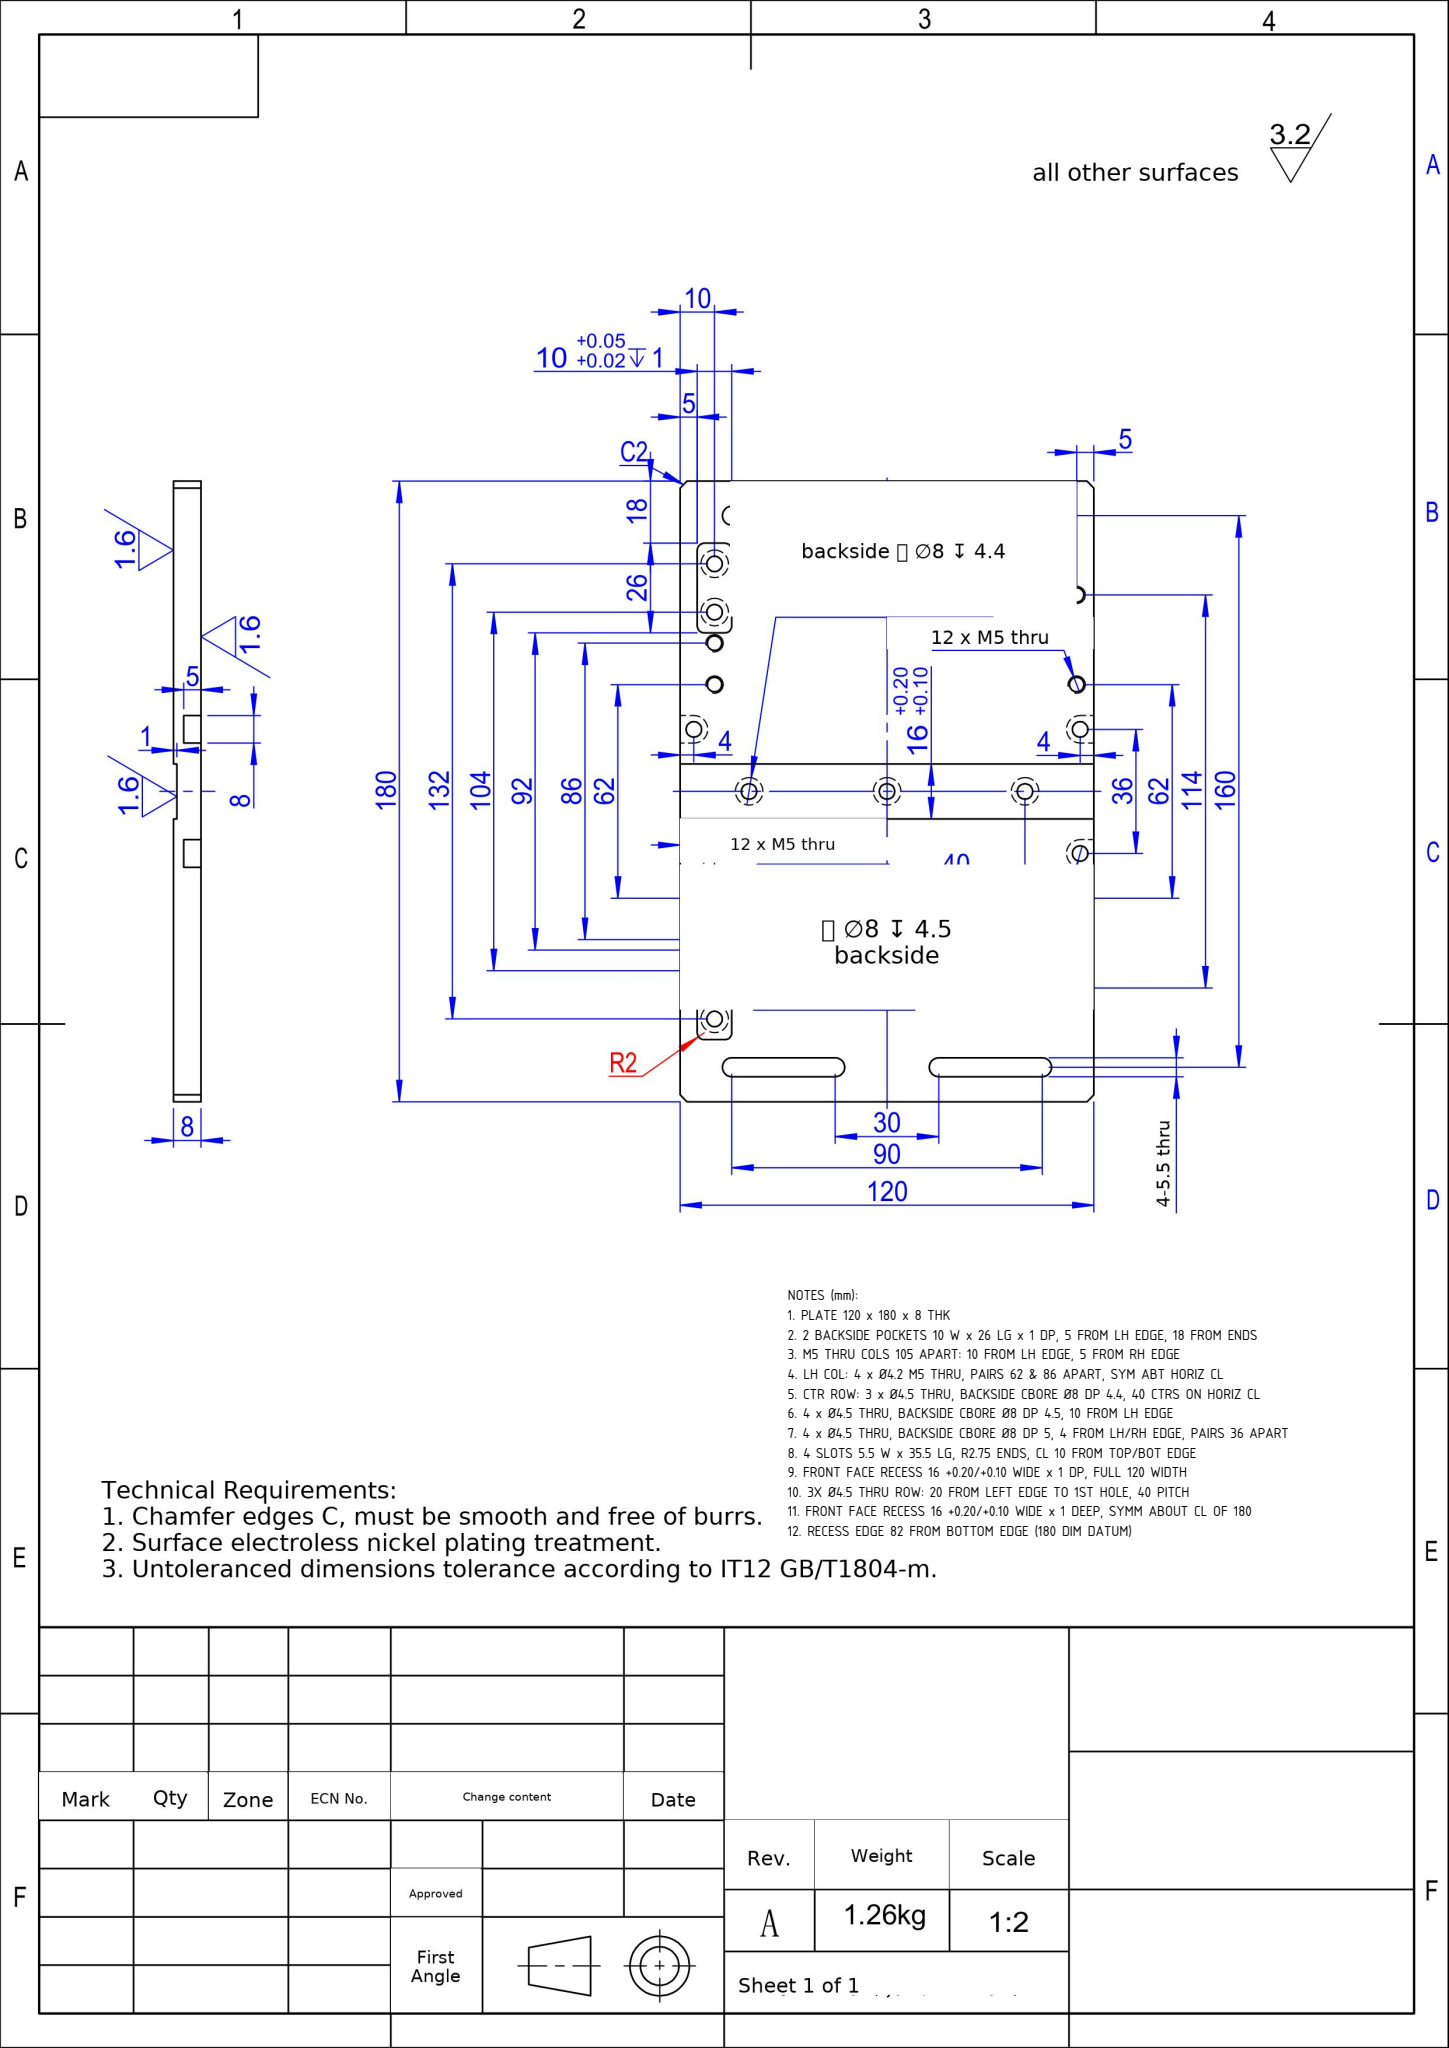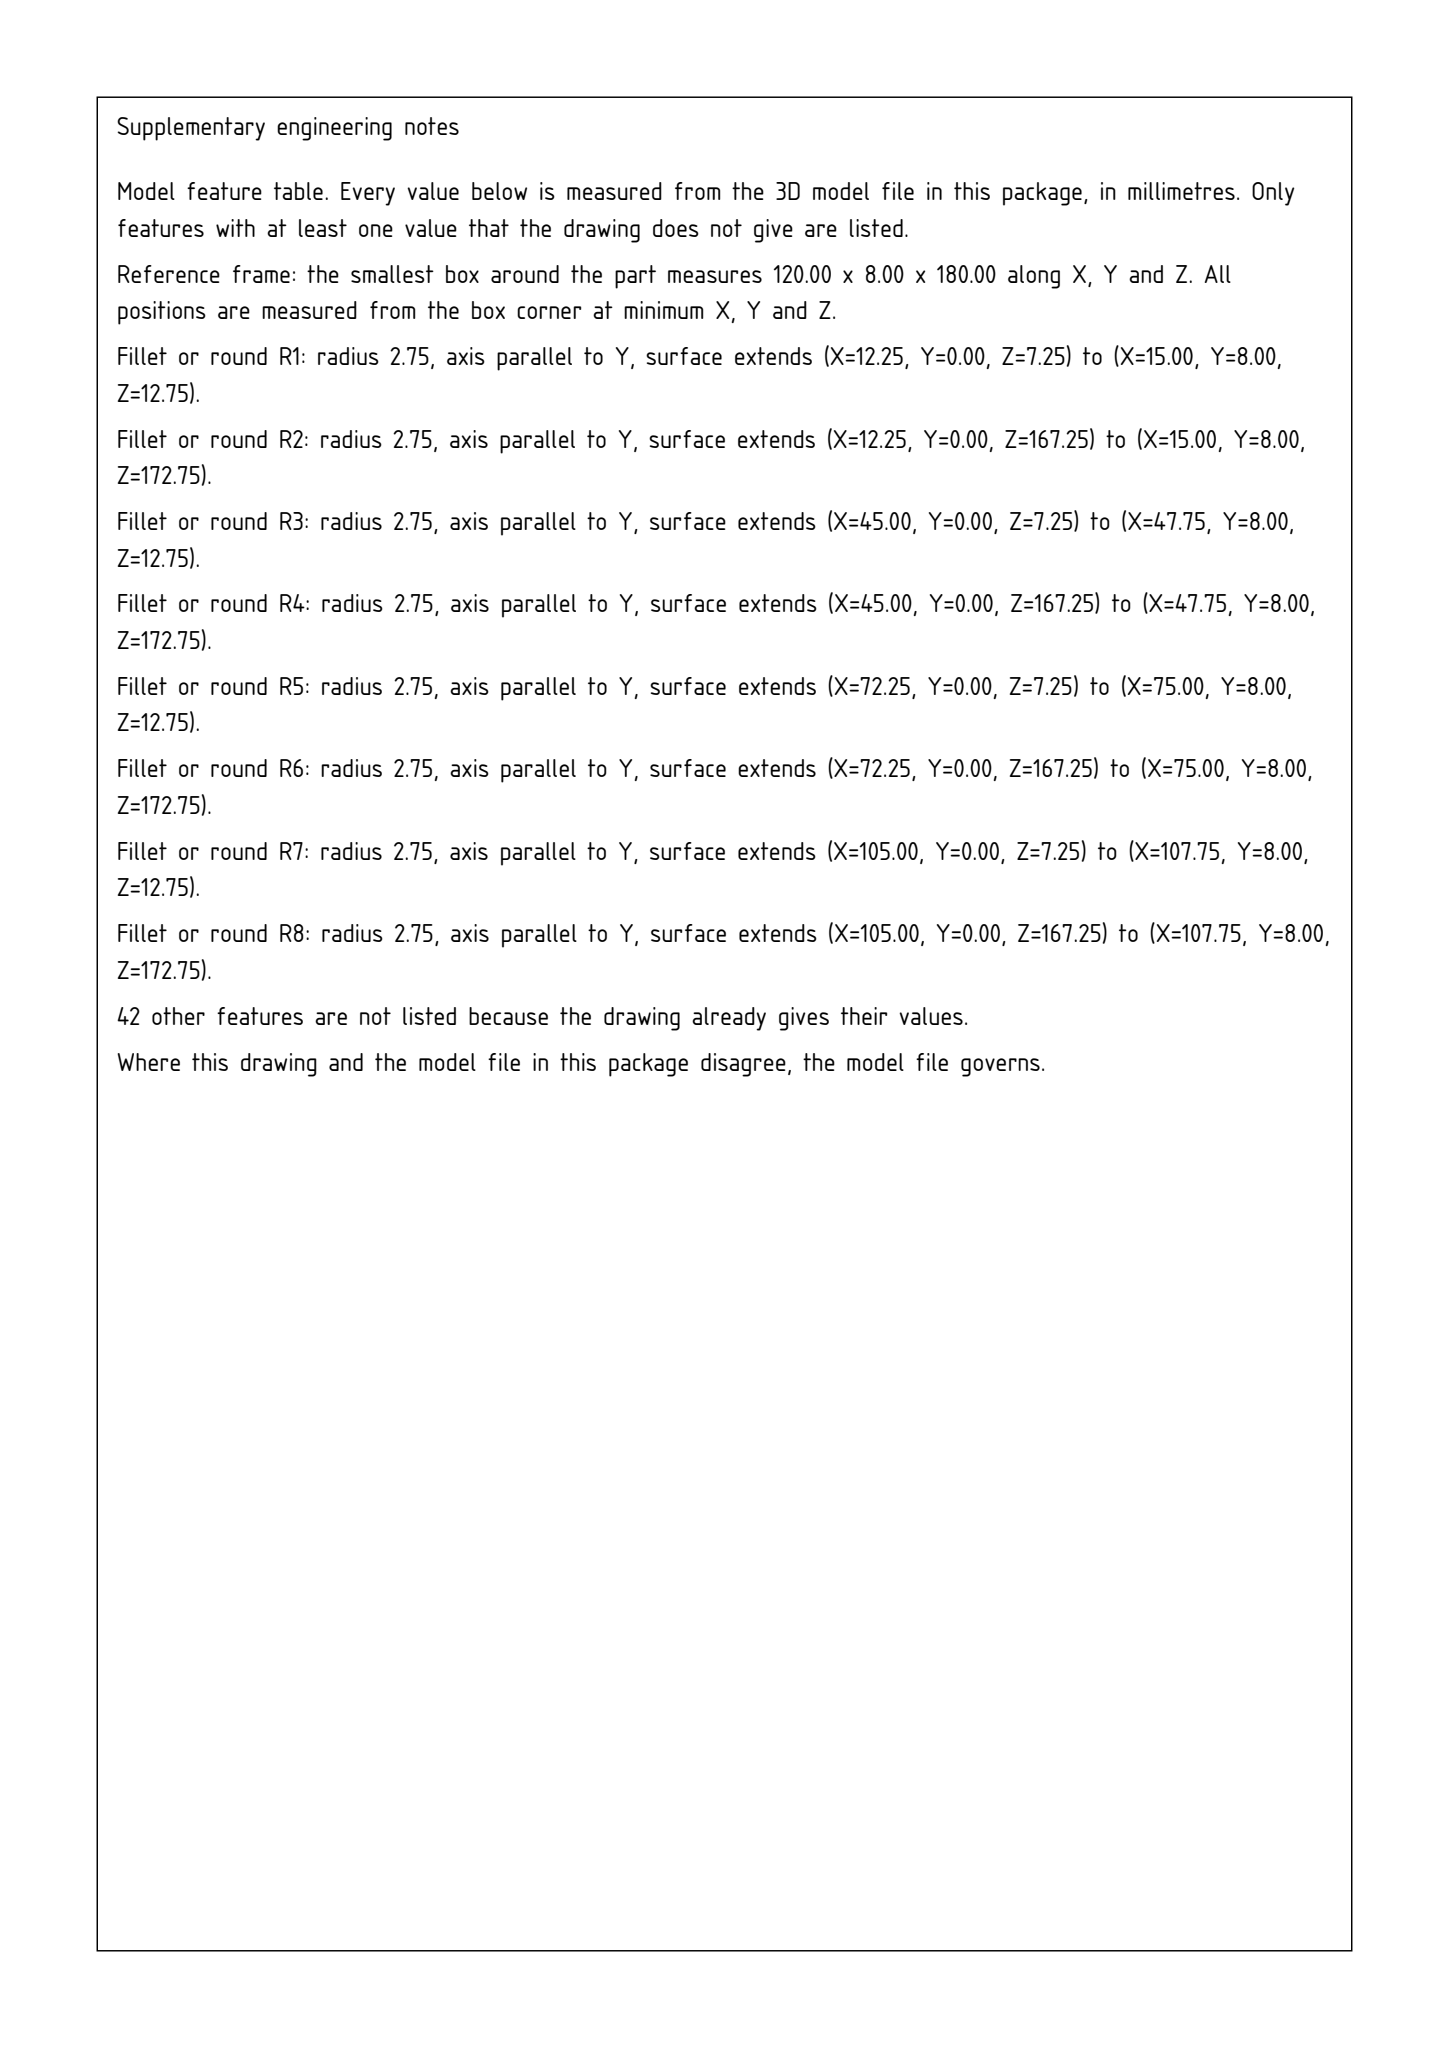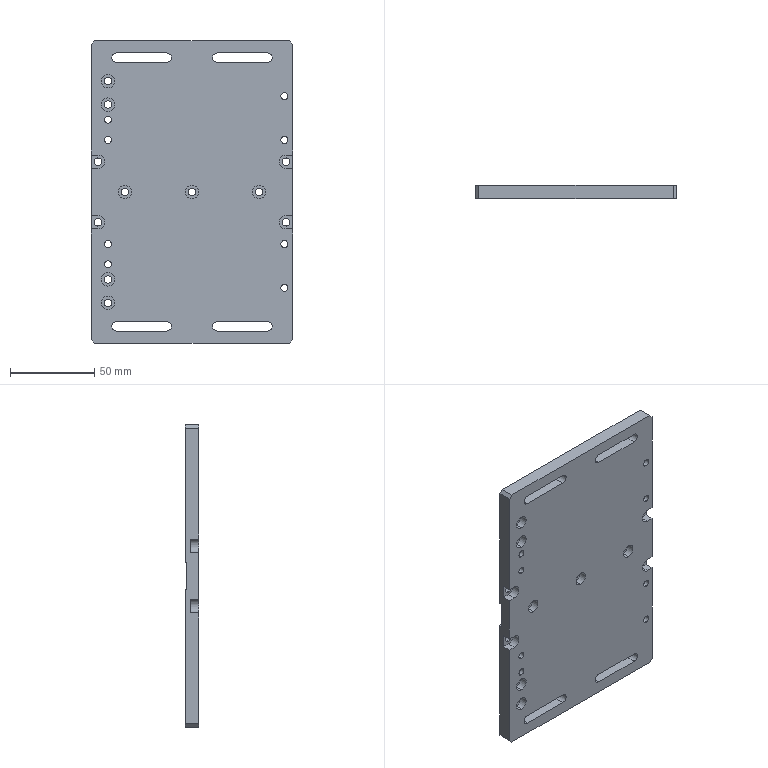Part | SolidWorks | mm | 1 solid | 123 faces | box 120 x 8 x 180 mm | volume 160191 mm3 | cylinder 72 | plane 51 | commonest cylinder face diameters 4.5 x22 8 x18 4.2 x16 4 x8 5.5 x8
Drawing notes:
PLATE 120 x 180 x 8 THK | from the solid: bbox_xyz 120 x 8 x 180
2 BACKSIDE POCKETS 10 W x 26 LG x 1 DP, 5 FROM LH EDGE, 18 FROM ENDS | from the solid: x planes 5 & 15 (10 wide); y 7.0 vs 8.0 face = 1 DP; z 18-44 & 136-162 (26 lg, 18 from ends)
M5 THRU COLS 105 APART: 10 FROM LH EDGE, 5 FROM RH EDGE | from the solid: Ø4.2 thru cols at x=10 and x=115; 115-10=105; 120-115=5
LH COL: 4 x Ø4.2 M5 THRU, PAIRS 62 & 86 APART, SYM ABT HORIZ CL | from the solid: Ø4.2 thru (len 8) at x=10, z=47/59/121/133; 59-121=62, 47-133=86, sym about z=90
CTR ROW: 3 x Ø4.5 THRU, BACKSIDE CBORE Ø8 DP 4.4, 40 CTRS ON HORIZ CL | from the solid: Ø4.5 at x=20,60,100 (40 spacing), z=90=180/2; Ø8 cbore len 4.4 same axes
4 x Ø4.5 THRU, BACKSIDE CBORE Ø8 DP 4.5, 10 FROM LH EDGE | from the solid: Ø4.5 y-holes at x=10, z=24,38,142,156 with Ø8 cbore len 4.5
4 x Ø4.5 THRU, BACKSIDE CBORE Ø8 DP 5, 4 FROM LH/RH EDGE, PAIRS 36 APART | from the solid: Ø4.5 at x=4 & 116, z=72 & 108 (36 apart, sym abt z=90); Ø8 cbore len 5
4 SLOTS 5.5 W x 35.5 LG, R2.75 ENDS, CL 10 FROM TOP/BOT EDGE | from the solid: Ø5.5 thru ends x=15/45 & 75/105 at z=10 and z=170; z planes 7.25/12.75 & 167.25/172.75
FRONT FACE RECESS 16 +0.20/+0.10 WIDE x 1 DP, FULL 120 WIDTH | from the solid: Z planes 82 & 98 (16 apart), Y plane 7.0 vs front face Y=8.0 -> 1 deep; spans X 0-120 (bbox width)
3X Ø4.5 THRU ROW: 20 FROM LEFT EDGE TO 1ST HOLE, 40 PITCH | from the solid: Ø4.5 holes at X=20, 60, 100 (Z=90); left edge X=0; middle hole on part CL X=60
FRONT FACE RECESS 16 +0.20/+0.10 WIDE x 1 DEEP, SYMM ABOUT CL OF 180 | from the solid: z-planes 82 & 98 bound 16 wide slot, centred at z=90 = 180/2; depth 1 (y 7.0 to 8.0), full 120 width
RECESS EDGE 82 FROM BOTTOM EDGE (180 DIM DATUM) | from the solid: z=82 and z=98 planes on 180 length from z=0 edge
build123d program:
from build123d import *

# Parameters (mm, degrees)
SKETCH1_W                                       = 120
SKETCH1_H                                       = 180
BOSS_EXTRUDE1_DEPTH                             = 8
SKETCH2_W                                       = 120
SKETCH2_H                                       = 16
CUT_EXTRUDE1_DEPTH                              = 1
M4_HEX_SOCKET_HEAD_CAP_SCREW_CBORE2_D           = 4.5
M4_HEX_SOCKET_HEAD_CAP_SCREW_CBORE2_CBORE_D     = 8
M4_HEX_SOCKET_HEAD_CAP_SCREW_CBORE2_CBORE_DEPTH = 4.4
M4_HEX_SOCKET_HEAD_CAP_SCREW_CBORE1_D           = 4.5
M4_HEX_SOCKET_HEAD_CAP_SCREW_CBORE1_CBORE_D     = 8
M4_HEX_SOCKET_HEAD_CAP_SCREW_CBORE1_CBORE_DEPTH = 4.5
SKETCH21_W                                      = 10
SKETCH21_H                                      = 26
CUT_EXTRUDE5_DEPTH                              = 1
FILLET2_R                                       = 2
CUT_EXTRUDE2_DEPTH                              = 109.462
FILLET2_OF_MIRROR1_R                            = 2
CHAMFER1_SIZE                                   = 2
MIRROR9_COPY_1_DEPTH                            = 109.462
LPATTERN3_COUNT                                 = 3
LPATTERN3_PITCH                                 = 40
M5_TAPPED_HOLE1_D                               = 4.2
M5_TAPPED_HOLE2_D                               = 4.2
M4_CLEARANCE_HOLE1_D                            = 4.5
CUT_EXTRUDE4_DEPTH                              = 5


with BuildPart() as part:
    # Sketch1 → Boss-Extrude1 (new body)
    with BuildSketch(Plane(origin=(0, 0, 0), x_dir=(1, 0, 0), z_dir=(0, 1, 0))):
        Rectangle(SKETCH1_W, SKETCH1_H)
    extrude(amount=BOSS_EXTRUDE1_DEPTH)

    # Sketch2 → Cut-Extrude1 (cut)
    with BuildSketch(Plane(origin=(0, 8, 0), x_dir=(1, 0, 0), z_dir=(0, 1, 0))):
        Rectangle(SKETCH2_W, SKETCH2_H)
    extrude(amount=-CUT_EXTRUDE1_DEPTH, mode=Mode.SUBTRACT)

    # M4 Hex Socket Head Cap Screw CBORE2 (through all)
    with Locations(Plane(origin=(-43.77, 0, -25.954), x_dir=(-1, 0, 0), z_dir=(0, -1, 0))):
        with Locations((-3.77, -25.954)):
            m4_hex_socket_head_cap_screw_cbore2 = CounterBoreHole(M4_HEX_SOCKET_HEAD_CAP_SCREW_CBORE2_D / 2, M4_HEX_SOCKET_HEAD_CAP_SCREW_CBORE2_CBORE_D / 2, M4_HEX_SOCKET_HEAD_CAP_SCREW_CBORE2_CBORE_DEPTH)

    # M4 Hex Socket Head Cap Screw CBORE1 (through all)
    with Locations(Plane.XZ):
        with Locations((-50, 66), (-50, 52)):
            m4_hex_socket_head_cap_screw_cbore1 = CounterBoreHole(M4_HEX_SOCKET_HEAD_CAP_SCREW_CBORE1_D / 2, M4_HEX_SOCKET_HEAD_CAP_SCREW_CBORE1_CBORE_D / 2, M4_HEX_SOCKET_HEAD_CAP_SCREW_CBORE1_CBORE_DEPTH)

    # Sketch21 → Cut-Extrude5 (cut)
    with BuildSketch(Plane(origin=(0, 8, 0), x_dir=(1, 0, 0), z_dir=(0, 1, 0))):
        with Locations((-50, -59)):
            Rectangle(SKETCH21_W, SKETCH21_H)
    cut_extrude5 = extrude(amount=-CUT_EXTRUDE5_DEPTH, mode=Mode.SUBTRACT)

    # Fillet2
    fillet2_edges = [part.edges().sort_by_distance(p)[0] for p in [
        (-55, 7.5, 72),
        (-55, 7.5, 46),
        (-45, 7.5, 46),
        (-45, 7.5, 72),
    ]]
    fillet(fillet2_edges, radius=FILLET2_R)

    # Sketch9 → Cut-Extrude2 (cut, through all)
    with BuildSketch(Plane(origin=(0, 8, 0), x_dir=(1, 0, 0), z_dir=(0, 1, 0))):
        with BuildLine():
            Line((15, -77.25), (45, -77.25))
            ThreePointArc((45, -77.25), (47.75, -80), (45, -82.75))
            Line((45, -82.75), (15, -82.75))
            ThreePointArc((15, -82.75), (12.25, -80), (15, -77.25))
        make_face()
    cut_extrude2 = extrude(amount=-CUT_EXTRUDE2_DEPTH, mode=Mode.SUBTRACT)

    # Mirror1: M4 Hex Socket Head Cap Screw CBORE1, Cut-Extrude5 across plane
    add(m4_hex_socket_head_cap_screw_cbore1.mirror(Plane.XY), mode=Mode.SUBTRACT)
    add(cut_extrude5.mirror(Plane.XY), mode=Mode.SUBTRACT)

    # Fillet2 of Mirror1
    fillet2_of_mirror1_edges = [part.edges().sort_by_distance(p)[0] for p in [
        (-55, 7.5, -72),
        (-55, 7.5, -46),
        (-45, 7.5, -46),
        (-45, 7.5, -72),
    ]]
    fillet(fillet2_of_mirror1_edges, radius=FILLET2_OF_MIRROR1_R)

    # Chamfer1
    chamfer1_edges = [part.edges().sort_by_distance(p)[0] for p in [
        (-60, 4, -90),
        (60, 4, -90),
        (60, 4, 90),
        (-60, 4, 90),
    ]]
    chamfer(chamfer1_edges, length=CHAMFER1_SIZE)

    # Mirror8: Cut-Extrude2 across plane
    add(cut_extrude2.mirror(Plane(origin=(0, 0, 0), x_dir=(0, 0, 1), z_dir=(1, 0, 0))), mode=Mode.SUBTRACT)

    # Mirror9: Cut-Extrude2 across plane
    add(cut_extrude2.mirror(Plane.XY), mode=Mode.SUBTRACT)

    # Mirror9 copy 1 sketch → Mirror9 copy 1 (cut, through all)
    with BuildSketch(Plane(origin=(0, 8, 0), x_dir=(-1, 0, 0), z_dir=(0, 1, 0))):
        with BuildLine():
            Line((15, -77.25), (45, -77.25))
            ThreePointArc((45, -77.25), (47.75, -80), (45, -82.75))
            Line((45, -82.75), (15, -82.75))
            ThreePointArc((15, -82.75), (12.25, -80), (15, -77.25))
        make_face()
    extrude(amount=-MIRROR9_COPY_1_DEPTH, mode=Mode.SUBTRACT)

    # LPattern3: M4 Hex Socket Head Cap Screw CBORE2 ×3
    with Locations(*[(i * LPATTERN3_PITCH, 0, 0) for i in range(1, LPATTERN3_COUNT)]):
        add(m4_hex_socket_head_cap_screw_cbore2, mode=Mode.SUBTRACT)

    # M5 Tapped Hole1 (through all)
    with Locations(Plane(origin=(0, 8, 0), x_dir=(-1, 0, 0), z_dir=(0, 1, 0))):
        with Locations((50, 31), (50, 43)):
            m5_tapped_hole1 = Hole(M5_TAPPED_HOLE1_D / 2)

    # M5 Tapped Hole2 (through all)
    with Locations(Plane(origin=(0, 8, 0), x_dir=(-1, 0, 0), z_dir=(0, 1, 0))):
        with Locations((-55, 31), (-55, 57)):
            m5_tapped_hole2 = Hole(M5_TAPPED_HOLE2_D / 2)

    # Mirror3: M5 Tapped Hole1, M5 Tapped Hole2 across plane
    add(m5_tapped_hole1.mirror(Plane.XY), mode=Mode.SUBTRACT)
    add(m5_tapped_hole2.mirror(Plane.XY), mode=Mode.SUBTRACT)

    # M4 Clearance Hole1 (through all)
    with Locations(Plane.XZ):
        with Locations((56, -18), (56, 18)):
            m4_clearance_hole1 = Hole(M4_CLEARANCE_HOLE1_D / 2)

    # Mirror5: M4 Clearance Hole1 across plane
    add(m4_clearance_hole1.mirror(Plane(origin=(0, 0, 0), x_dir=(0, 0, 1), z_dir=(1, 0, 0))), mode=Mode.SUBTRACT)

    # Sketch17 → Cut-Extrude4 (cut)
    with BuildSketch(Plane.XZ):
        with BuildLine():
            Line((56, 22), (60, 22))
            Line((60, 22), (60, 14))
            Line((60, 14), (56, 14))
            ThreePointArc((56, 14), (52, 18), (56, 22))
        make_face()
        with BuildLine():
            Line((-56, 22), (-60, 22))
            Line((-60, 22), (-60, 14))
            Line((-60, 14), (-56, 14))
            ThreePointArc((-56, 14), (-52, 18), (-56, 22))
        make_face()
    cut_extrude4 = extrude(amount=-CUT_EXTRUDE4_DEPTH, mode=Mode.SUBTRACT)

    # Mirror6: Cut-Extrude4 across plane
    add(cut_extrude4.mirror(Plane.XY), mode=Mode.SUBTRACT)


solid = part.part